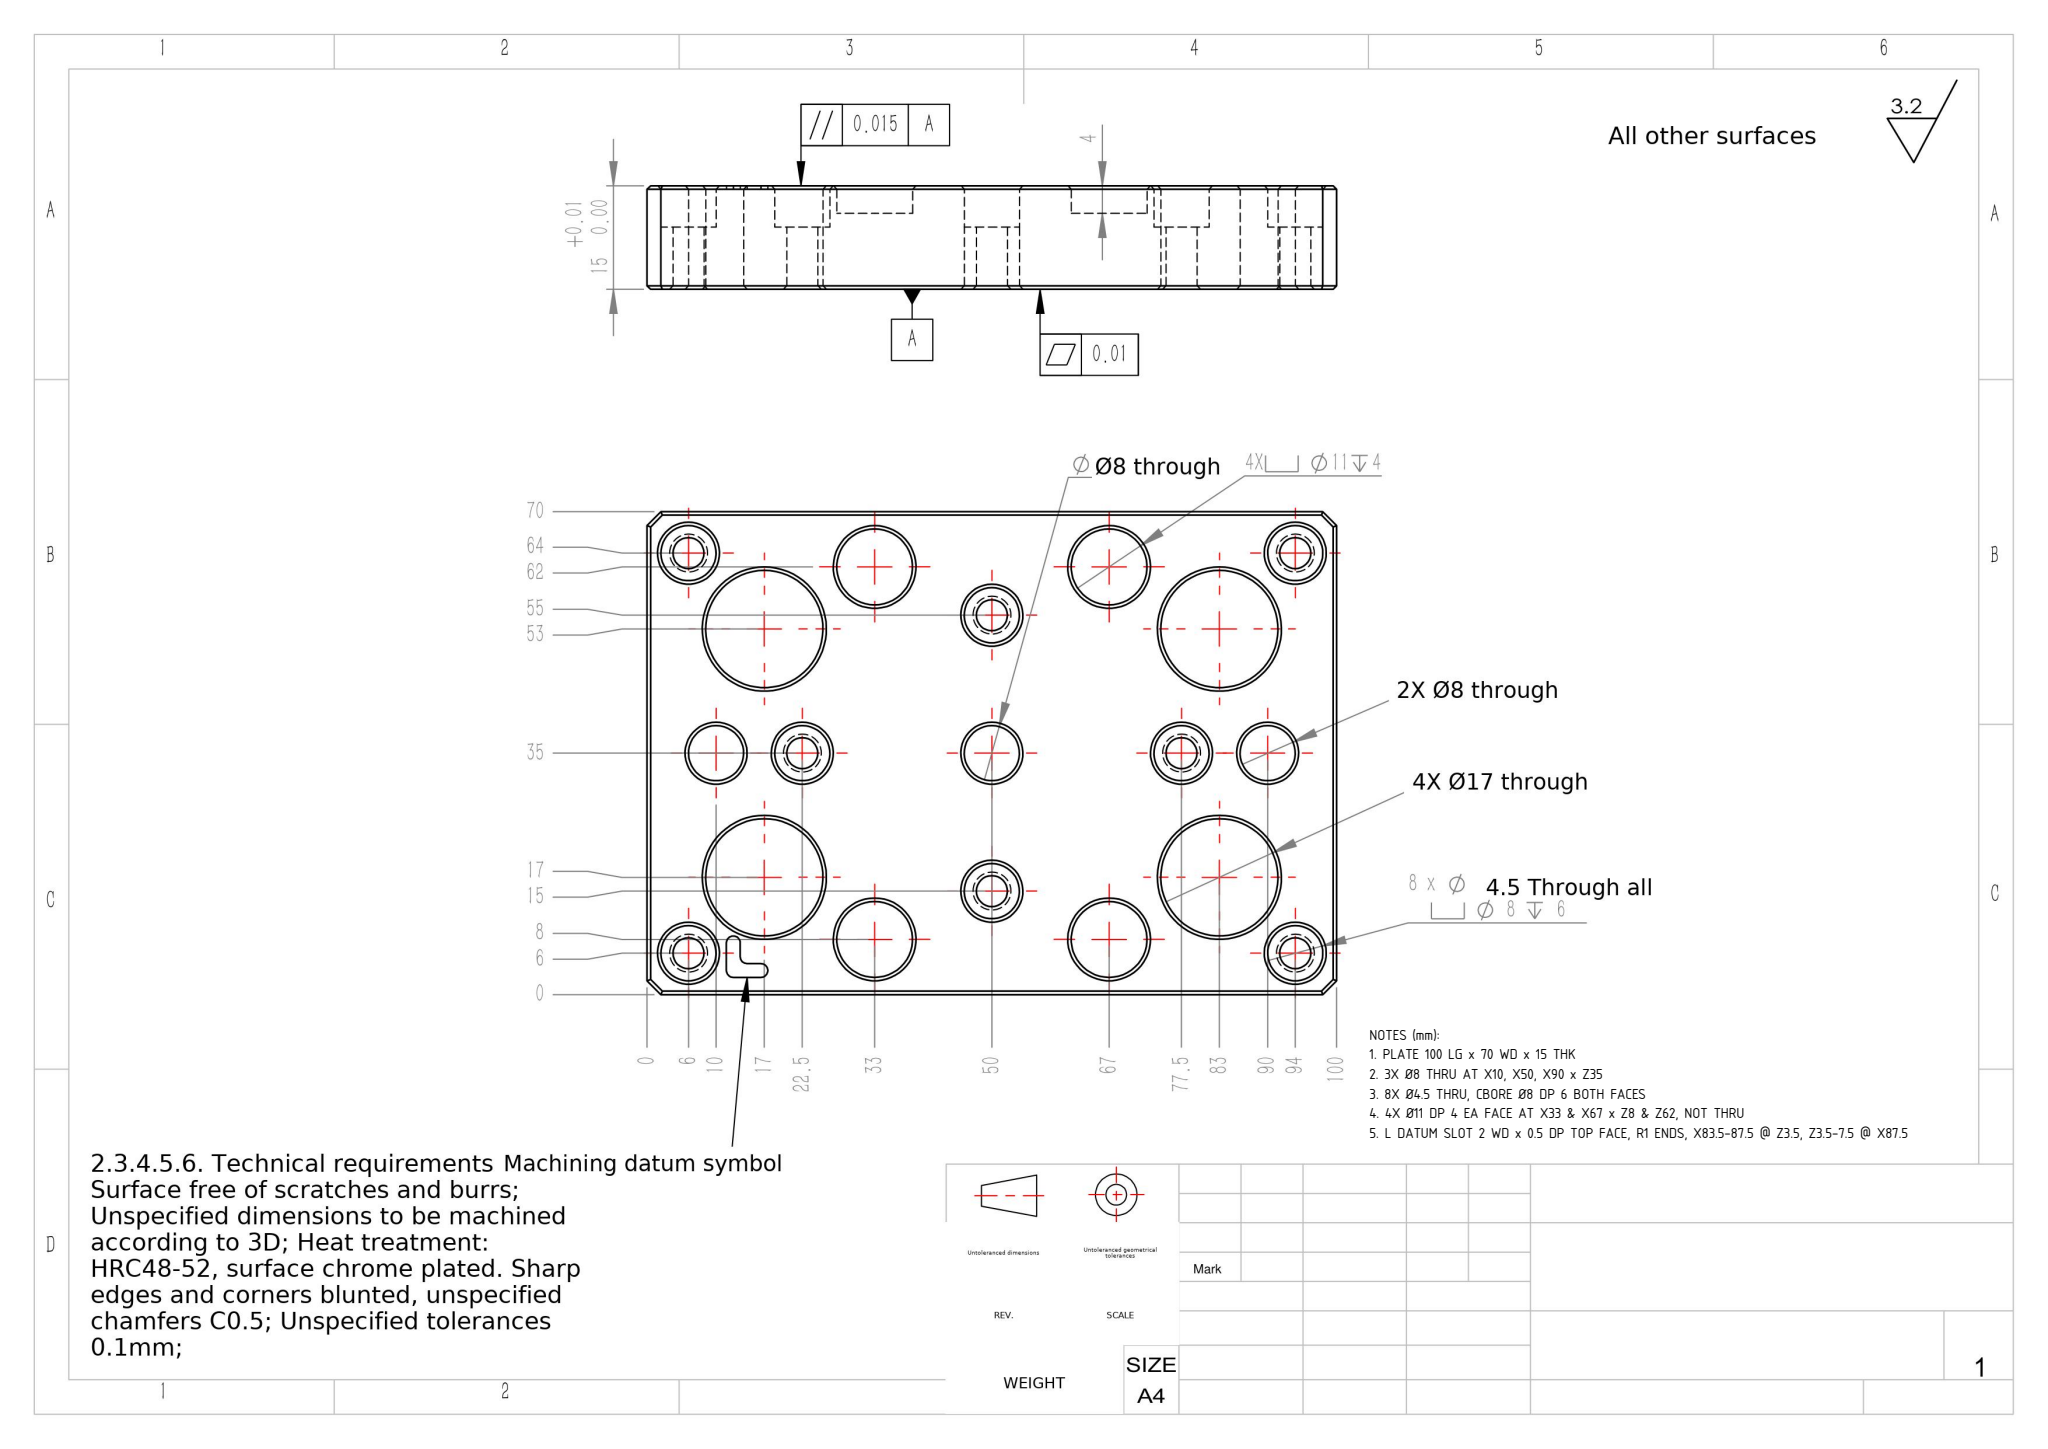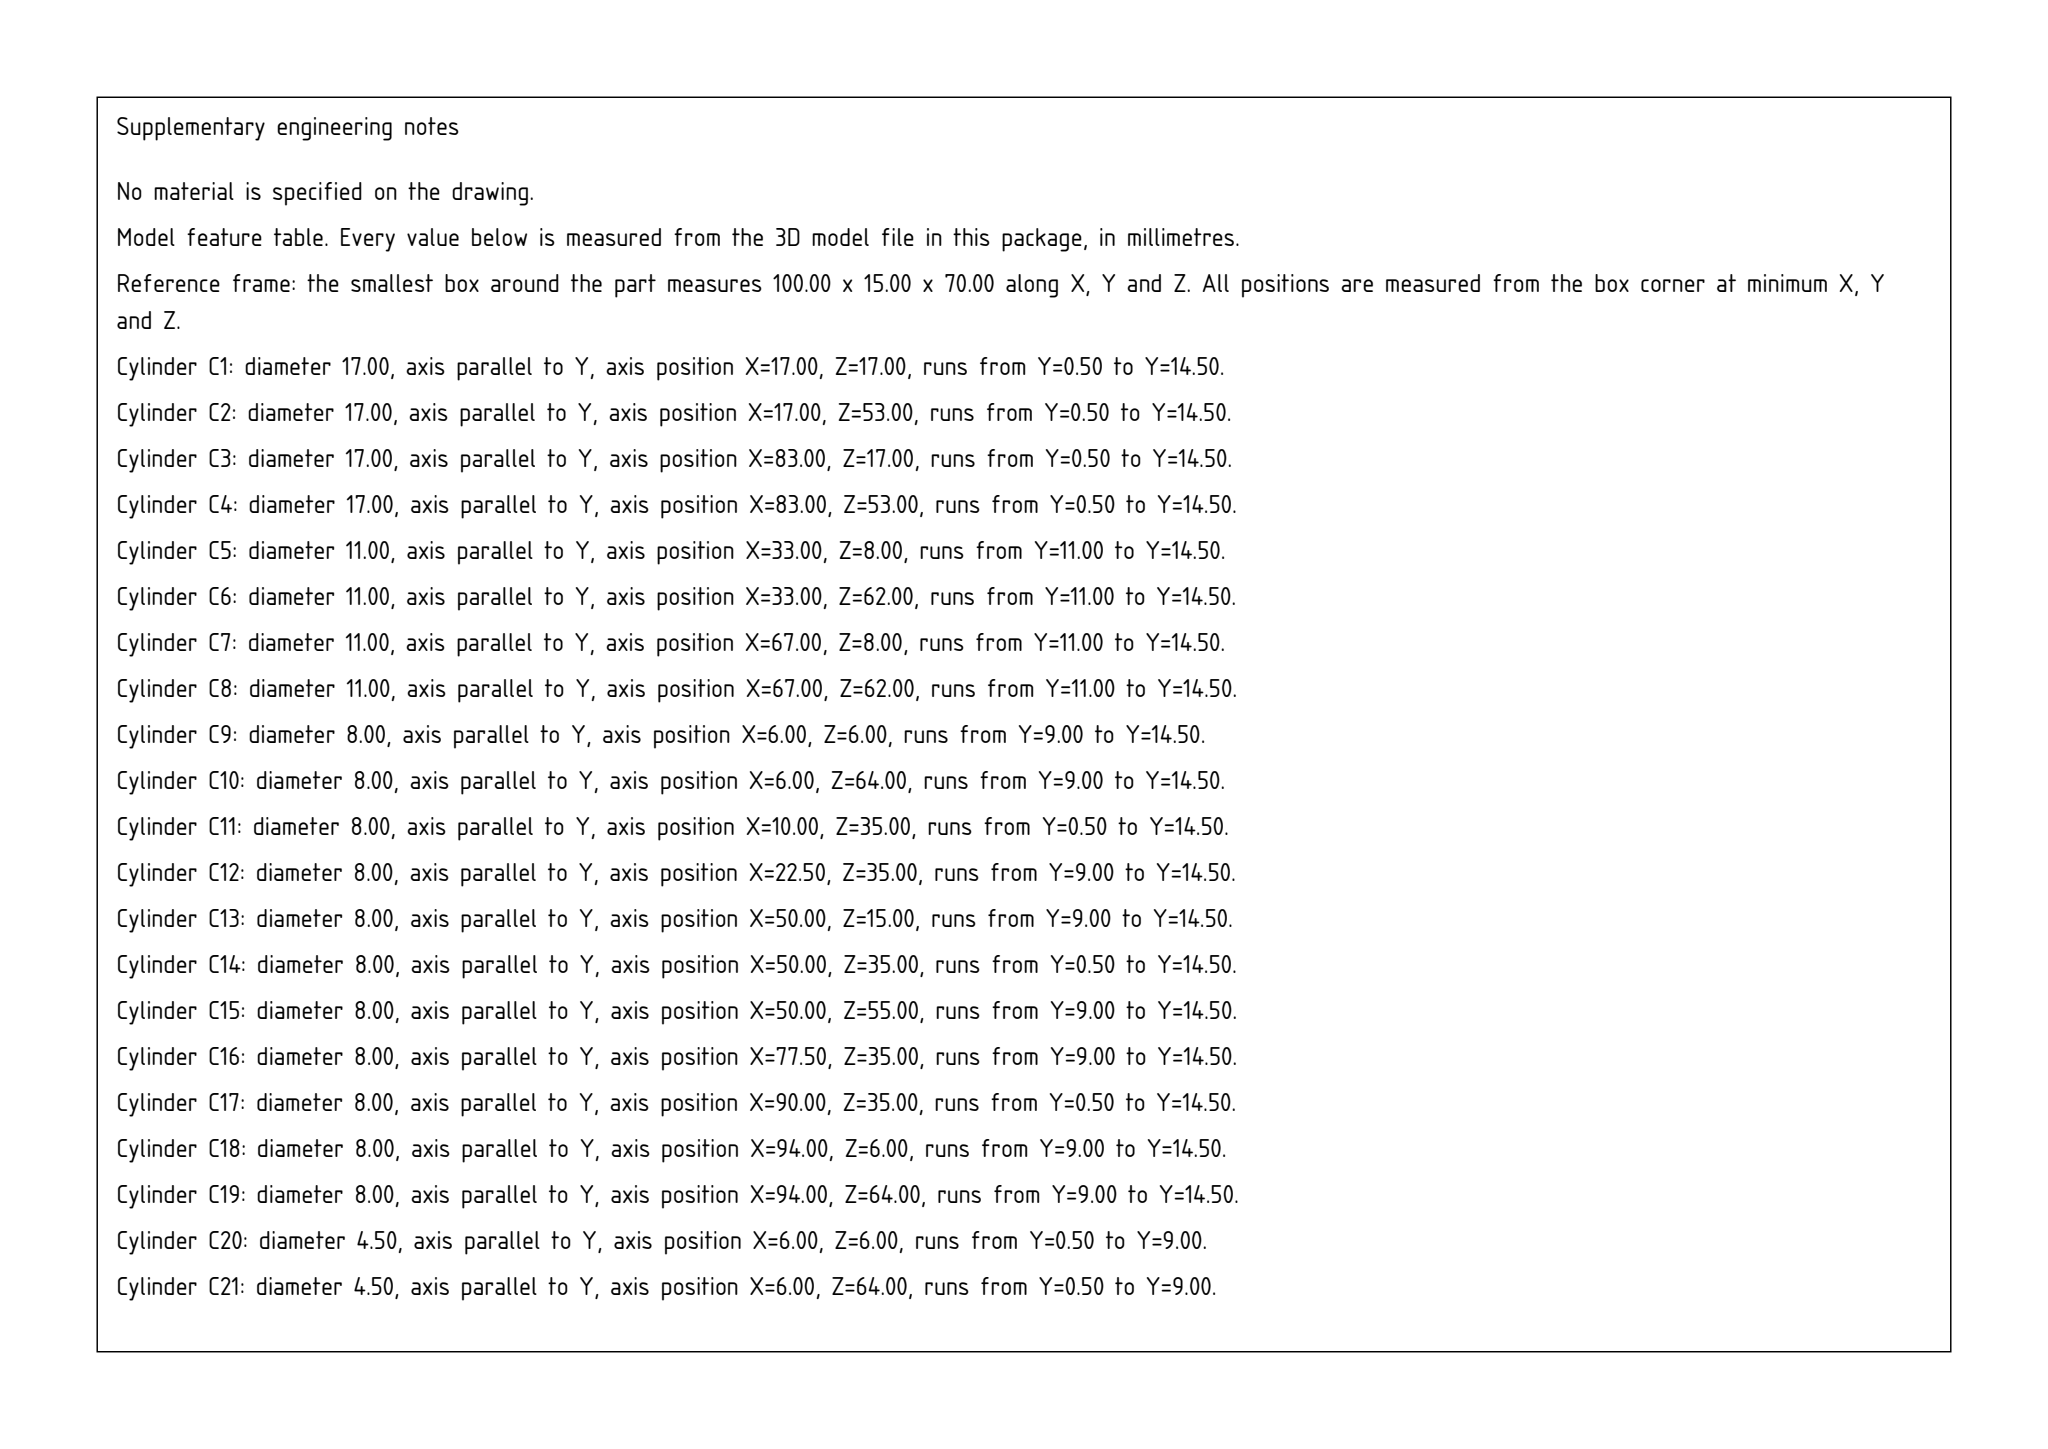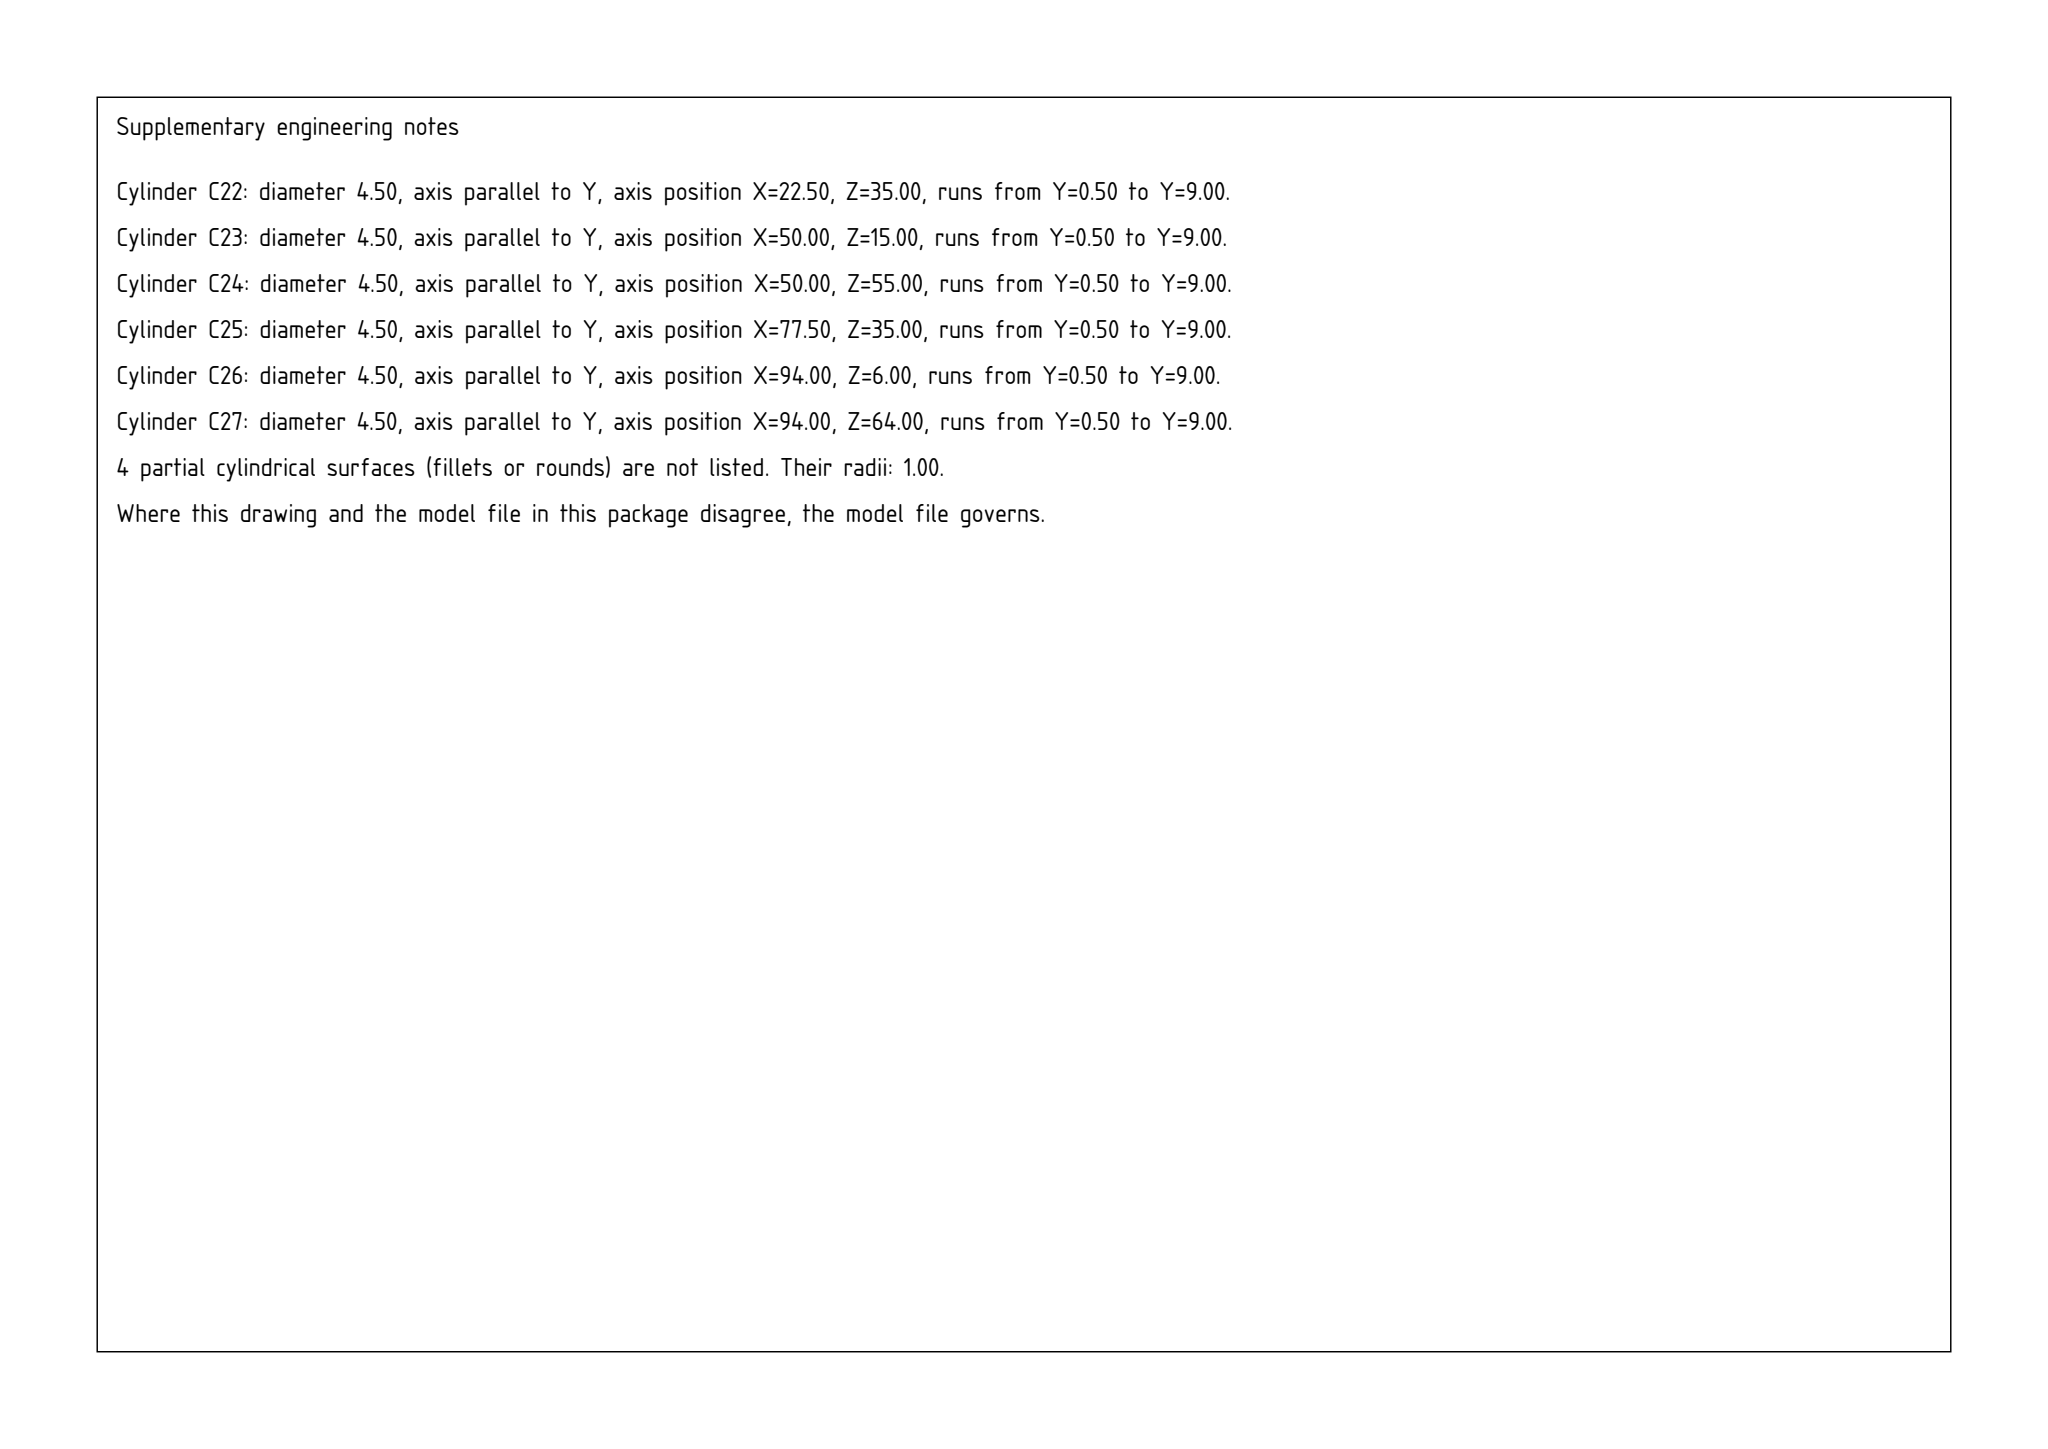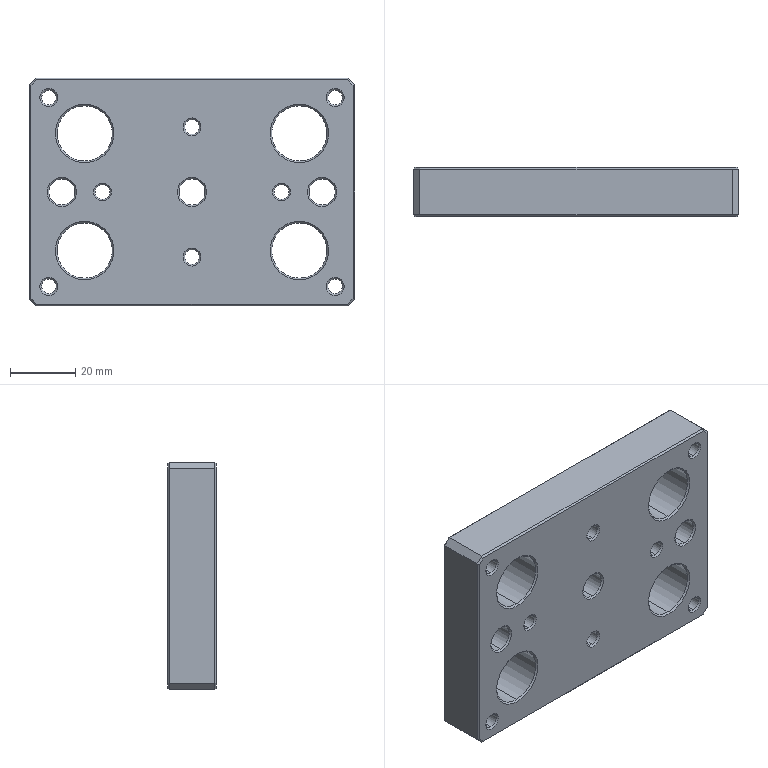Part | SolidWorks | mm | 1 solid | 171 faces | box 100 x 15 x 70 mm | volume 83694 mm3 | cone 68 | cylinder 60 | plane 43 | commonest cylinder face diameters 8 x22 4.5 x16 17 x8 11 x8 2 x6
Drawing notes:
PLATE 100 LG x 70 WD x 15 THK | from the solid: bbox_xyz [100.0, 15.0, 70.0]
3X Ø8 THRU AT X10, X50, X90 x Z35 | from the solid: Cyl dia 8.0, axis y, L=14.0 (15 thk less chamfers) at (10,35),(50,35),(90,35)
8X Ø4.5 THRU, CBORE Ø8 DP 6 BOTH FACES | from the solid: Ø4.5 L=8.5 x2 and Ø8 L=5.5 x2 at 8 posns (6,6),(6,64),(22.5,35),(50,15),(50,55),(77.5,35),(94,6),(94,64); plane y=9.0 count 8
4X Ø11 DP 4 EA FACE AT X33 & X67 x Z8 & Z62, NOT THRU | from the solid: Ø11 cyl L=3.5 +0.5 chf, count 2 per locn at (33,8),(33,62),(67,8),(67,62); plane y=11.0 (15-11=4)
L DATUM SLOT 2 WD x 0.5 DP TOP FACE, R1 ENDS, X83.5-87.5 @ Z3.5, Z3.5-7.5 @ X87.5 | from the solid: Ø2 cyls L=0.5 at (83.5,3.5),(87.5,3.5),(87.5,7.5), R1 corner (85.5,5.5); y-planes 14.5/15, x-planes 86.5/88.5, z-planes 2.5/4.5